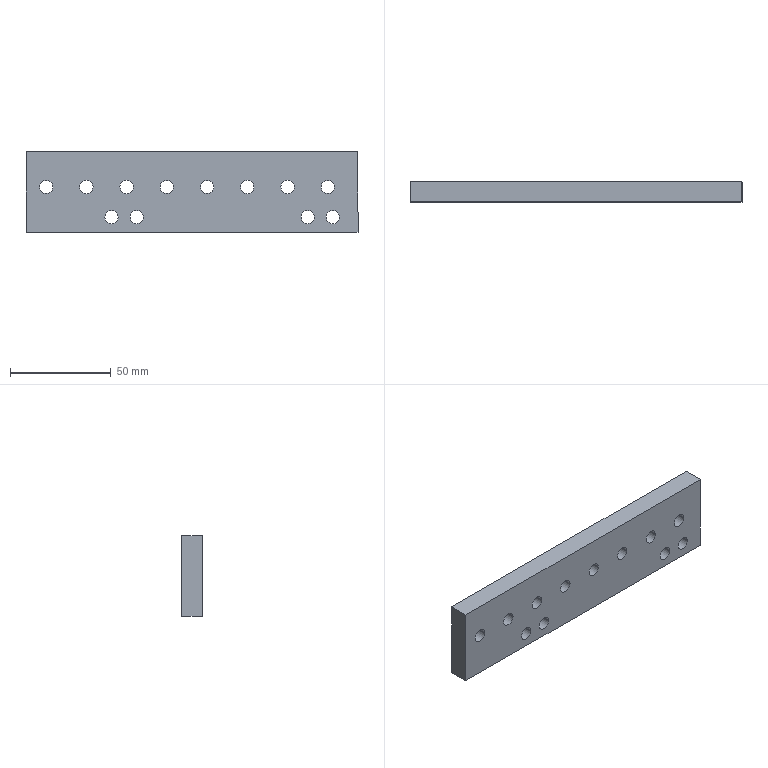Component | SolidWorks | CTM-HVS-42-02-31-4 | 1 solid | 30 faces | box 165 x 10 x 40 mm | volume 61895 mm3 | cylinder 24 | plane 6 | commonest cylinder face diameters 6.6 x24 | material Bakelite
build123d program:
from build123d import *

# Parameters (mm, degrees)
SKETCH1_W          = 185
SKETCH1_H          = 40
EXTRUDE1_DEPTH     = 10
CUT_EXTRUDE1_REACH = 152.748
SKETCH2_R          = 3.3
LPATTERN1_COUNT    = 9
LPATTERN1_PITCH    = 20
SKETCH6_W          = 20
SKETCH6_H          = 40
CUT_EXTRUDE3_DEPTH = 10


with BuildPart() as part:
    # Sketch1 → Extrude1 (new body)
    with BuildSketch(Plane.XY):
        with Locations((52.5, -20)):
            Rectangle(SKETCH1_W, SKETCH1_H)
    extrude(amount=EXTRUDE1_DEPTH)

    # Sketch2 → Cut-Extrude1 (cut, up to next)
    with BuildSketch(Plane.XY.offset(10), mode=Mode.PRIVATE) as cut_extrude1_sk1:
        with Locations((-15, -7.5)):
            Circle(SKETCH2_R)
    cut_extrude1_tool1 = extrude(cut_extrude1_sk1.sketch, amount=-CUT_EXTRUDE1_REACH, mode=Mode.PRIVATE) & part.part
    # Sketch2 → Cut-Extrude1 (cut, up to next)
    with BuildSketch(Plane.XY.offset(10), mode=Mode.PRIVATE) as cut_extrude1_sk2:
        with Locations((70, -7.5)):
            Circle(SKETCH2_R)
    cut_extrude1_tool2 = extrude(cut_extrude1_sk2.sketch, amount=-CUT_EXTRUDE1_REACH, mode=Mode.PRIVATE) & part.part
    # Sketch2 → Cut-Extrude1 (cut, up to next)
    with BuildSketch(Plane.XY.offset(10), mode=Mode.PRIVATE) as cut_extrude1_sk3:
        with Locations((-27.5, -7.5)):
            Circle(SKETCH2_R)
    cut_extrude1_tool3 = extrude(cut_extrude1_sk3.sketch, amount=-CUT_EXTRUDE1_REACH, mode=Mode.PRIVATE) & part.part
    # Sketch2 → Cut-Extrude1 (cut, up to next)
    with BuildSketch(Plane.XY.offset(10), mode=Mode.PRIVATE) as cut_extrude1_sk4:
        with Locations((82.5, -7.5)):
            Circle(SKETCH2_R)
    cut_extrude1_tool4 = extrude(cut_extrude1_sk4.sketch, amount=-CUT_EXTRUDE1_REACH, mode=Mode.PRIVATE) & part.part
    add(cut_extrude1_tool1.solids().sort_by_distance((-15, -7.5, 10))[0], mode=Mode.SUBTRACT)
    add(cut_extrude1_tool2.solids().sort_by_distance((70, -7.5, 10))[0], mode=Mode.SUBTRACT)
    add(cut_extrude1_tool3.solids().sort_by_distance((-27.5, -7.5, 10))[0], mode=Mode.SUBTRACT)
    add(cut_extrude1_tool4.solids().sort_by_distance((82.5, -7.5, 10))[0], mode=Mode.SUBTRACT)

    # Sketch4 → M6 Clearance Hole1 (revolve, cut)
    with BuildSketch(Plane(origin=(-25, -22.5, 10), x_dir=(0, -1, 0), z_dir=(1, 0, 0))):
        Polygon((0, 0), (0, 31.983), (3.3, 30), (3.3, 0), align=None)
    m6_clearance_hole1 = revolve(axis=Axis((-25, -22.5, 16.35), (0, 0, -1)), mode=Mode.SUBTRACT)

    # LPattern1: M6 Clearance Hole1 ×9
    with Locations(*[(i * LPATTERN1_PITCH, 0, 0) for i in range(1, LPATTERN1_COUNT)]):
        add(m6_clearance_hole1, mode=Mode.SUBTRACT)

    # Sketch6 → Cut-Extrude3 (cut)
    with BuildSketch(Plane.XY.offset(10)):
        with Locations((135, -20)):
            Rectangle(SKETCH6_W, SKETCH6_H)
    extrude(amount=-CUT_EXTRUDE3_DEPTH, mode=Mode.SUBTRACT)


solid = part.part

# Placed as in the assembly
solid = solid.moved(Location((275.193, -64.557, -7.5), (90, 0, -180)))
STEP:
#1=COLOUR_RGB('',0.7922,0.8196,0.9333);
#2=FILL_AREA_STYLE_COLOUR('',#1);
#3=FILL_AREA_STYLE('',(#2));
#4=SURFACE_STYLE_FILL_AREA(#3);
#5=SURFACE_SIDE_STYLE('',(#4));
#6=SURFACE_STYLE_USAGE(.BOTH.,#5);
#7=PRESENTATION_STYLE_ASSIGNMENT((#6));
#8=CARTESIAN_POINT('',(6.177,-2.542,0.5906));
#9=VERTEX_POINT('',#8);
#10=CARTESIAN_POINT('',(6.437,-2.542,0.5906));
#11=VERTEX_POINT('',#10);
#12=CARTESIAN_POINT('',(6.307,-2.542,0.5906));
#13=DIRECTION('',(-0.,1.,-0.));
#14=DIRECTION('',(1.,0.,0.));
#15=AXIS2_PLACEMENT_3D('',#12,#13,#14);
#16=CIRCLE('',#15,0.1299);
#17=EDGE_CURVE('',#9,#11,#16,.T.);
#18=ORIENTED_EDGE('',*,*,#17,.T.);
#19=CARTESIAN_POINT('',(6.437,-2.935,0.5906));
#20=VERTEX_POINT('',#19);
#21=CARTESIAN_POINT('',(6.437,-2.935,0.5906));
#22=DIRECTION('',(0.,-1.,0.));
#23=VECTOR('',#22,39.37);
#24=LINE('',#21,#23);
#25=EDGE_CURVE('',#11,#20,#24,.T.);
#26=ORIENTED_EDGE('',*,*,#25,.T.);
#27=CARTESIAN_POINT('',(6.177,-2.935,0.5906));
#28=VERTEX_POINT('',#27);
#29=CARTESIAN_POINT('',(6.307,-2.935,0.5906));
#30=DIRECTION('',(0.,-1.,0.));
#31=DIRECTION('',(-1.,0.,-0.));
#32=AXIS2_PLACEMENT_3D('',#29,#30,#31);
#33=CIRCLE('',#32,0.1299);
#34=EDGE_CURVE('',#20,#28,#33,.T.);
#35=ORIENTED_EDGE('',*,*,#34,.T.);
#36=CARTESIAN_POINT('',(6.177,-2.935,0.5906));
#37=DIRECTION('',(0.,-1.,0.));
#38=VECTOR('',#37,39.37);
#39=LINE('',#36,#38);
#40=EDGE_CURVE('',#9,#28,#39,.T.);
#41=ORIENTED_EDGE('',*,*,#40,.F.);
#42=EDGE_LOOP('',(#18,#26,#35,#41));
#43=FACE_OUTER_BOUND('',#42,.T.);
#44=CARTESIAN_POINT('',(6.307,-2.935,0.5906));
#45=DIRECTION('',(0.,-1.,0.));
#46=DIRECTION('',(-1.,0.,-0.));
#47=AXIS2_PLACEMENT_3D('',#44,#45,#46);
#48=CYLINDRICAL_SURFACE('',#47,0.1299);
#49=ADVANCED_FACE('',(#43),#48,.F.);
#50=CARTESIAN_POINT('',(6.964,-2.542,0.5906));
#51=VERTEX_POINT('',#50);
#52=CARTESIAN_POINT('',(7.224,-2.542,0.5906));
#53=VERTEX_POINT('',#52);
#54=CARTESIAN_POINT('',(7.094,-2.542,0.5906));
#55=DIRECTION('',(-0.,1.,-0.));
#56=DIRECTION('',(1.,0.,0.));
#57=AXIS2_PLACEMENT_3D('',#54,#55,#56);
#58=CIRCLE('',#57,0.1299);
#59=EDGE_CURVE('',#51,#53,#58,.T.);
#60=ORIENTED_EDGE('',*,*,#59,.T.);
#61=CARTESIAN_POINT('',(7.224,-2.935,0.5906));
#62=VERTEX_POINT('',#61);
#63=CARTESIAN_POINT('',(7.224,-2.935,0.5906));
#64=DIRECTION('',(0.,-1.,0.));
#65=VECTOR('',#64,39.37);
#66=LINE('',#63,#65);
#67=EDGE_CURVE('',#53,#62,#66,.T.);
#68=ORIENTED_EDGE('',*,*,#67,.T.);
#69=CARTESIAN_POINT('',(6.964,-2.935,0.5906));
#70=VERTEX_POINT('',#69);
#71=CARTESIAN_POINT('',(7.094,-2.935,0.5906));
#72=DIRECTION('',(0.,-1.,0.));
#73=DIRECTION('',(-1.,0.,-0.));
#74=AXIS2_PLACEMENT_3D('',#71,#72,#73);
#75=CIRCLE('',#74,0.1299);
#76=EDGE_CURVE('',#62,#70,#75,.T.);
#77=ORIENTED_EDGE('',*,*,#76,.T.);
#78=CARTESIAN_POINT('',(6.964,-2.935,0.5906));
#79=DIRECTION('',(0.,-1.,0.));
#80=VECTOR('',#79,39.37);
#81=LINE('',#78,#80);
#82=EDGE_CURVE('',#51,#70,#81,.T.);
#83=ORIENTED_EDGE('',*,*,#82,.F.);
#84=EDGE_LOOP('',(#60,#68,#77,#83));
#85=FACE_OUTER_BOUND('',#84,.T.);
#86=CARTESIAN_POINT('',(7.094,-2.935,0.5906));
#87=DIRECTION('',(0.,-1.,0.));
#88=DIRECTION('',(-1.,0.,-0.));
#89=AXIS2_PLACEMENT_3D('',#86,#87,#88);
#90=CYLINDRICAL_SURFACE('',#89,0.1299);
#91=ADVANCED_FACE('',(#85),#90,.F.);
#92=CARTESIAN_POINT('',(7.752,-2.542,0.5906));
#93=VERTEX_POINT('',#92);
#94=CARTESIAN_POINT('',(8.012,-2.542,0.5906));
#95=VERTEX_POINT('',#94);
#96=CARTESIAN_POINT('',(7.882,-2.542,0.5906));
#97=DIRECTION('',(-0.,1.,-0.));
#98=DIRECTION('',(1.,0.,0.));
#99=AXIS2_PLACEMENT_3D('',#96,#97,#98);
#100=CIRCLE('',#99,0.1299);
#101=EDGE_CURVE('',#93,#95,#100,.T.);
#102=ORIENTED_EDGE('',*,*,#101,.T.);
#103=CARTESIAN_POINT('',(8.012,-2.935,0.5906));
#104=VERTEX_POINT('',#103);
#105=CARTESIAN_POINT('',(8.012,-2.935,0.5906));
#106=DIRECTION('',(0.,-1.,0.));
#107=VECTOR('',#106,39.37);
#108=LINE('',#105,#107);
#109=EDGE_CURVE('',#95,#104,#108,.T.);
#110=ORIENTED_EDGE('',*,*,#109,.T.);
#111=CARTESIAN_POINT('',(7.752,-2.935,0.5906));
#112=VERTEX_POINT('',#111);
#113=CARTESIAN_POINT('',(7.882,-2.935,0.5906));
#114=DIRECTION('',(0.,-1.,0.));
#115=DIRECTION('',(-1.,0.,-0.));
#116=AXIS2_PLACEMENT_3D('',#113,#114,#115);
#117=CIRCLE('',#116,0.1299);
#118=EDGE_CURVE('',#104,#112,#117,.T.);
#119=ORIENTED_EDGE('',*,*,#118,.T.);
#120=CARTESIAN_POINT('',(7.752,-2.935,0.5906));
#121=DIRECTION('',(0.,-1.,0.));
#122=VECTOR('',#121,39.37);
#123=LINE('',#120,#122);
#124=EDGE_CURVE('',#93,#112,#123,.T.);
#125=ORIENTED_EDGE('',*,*,#124,.F.);
#126=EDGE_LOOP('',(#102,#110,#119,#125));
#127=FACE_OUTER_BOUND('',#126,.T.);
#128=CARTESIAN_POINT('',(7.882,-2.935,0.5906));
#129=DIRECTION('',(0.,-1.,0.));
#130=DIRECTION('',(-1.,0.,-0.));
#131=AXIS2_PLACEMENT_3D('',#128,#129,#130);
#132=CYLINDRICAL_SURFACE('',#131,0.1299);
#133=ADVANCED_FACE('',(#127),#132,.F.);
#134=CARTESIAN_POINT('',(8.539,-2.542,0.5906));
#135=VERTEX_POINT('',#134);
#136=CARTESIAN_POINT('',(8.799,-2.542,0.5906));
#137=VERTEX_POINT('',#136);
#138=CARTESIAN_POINT('',(8.669,-2.542,0.5906));
#139=DIRECTION('',(-0.,1.,-0.));
#140=DIRECTION('',(1.,0.,0.));
#141=AXIS2_PLACEMENT_3D('',#138,#139,#140);
#142=CIRCLE('',#141,0.1299);
#143=EDGE_CURVE('',#135,#137,#142,.T.);
#144=ORIENTED_EDGE('',*,*,#143,.T.);
#145=CARTESIAN_POINT('',(8.799,-2.935,0.5906));
#146=VERTEX_POINT('',#145);
#147=CARTESIAN_POINT('',(8.799,-2.935,0.5906));
#148=DIRECTION('',(0.,-1.,0.));
#149=VECTOR('',#148,39.37);
#150=LINE('',#147,#149);
#151=EDGE_CURVE('',#137,#146,#150,.T.);
#152=ORIENTED_EDGE('',*,*,#151,.T.);
#153=CARTESIAN_POINT('',(8.539,-2.935,0.5906));
#154=VERTEX_POINT('',#153);
#155=CARTESIAN_POINT('',(8.669,-2.935,0.5906));
#156=DIRECTION('',(0.,-1.,0.));
#157=DIRECTION('',(-1.,0.,-0.));
#158=AXIS2_PLACEMENT_3D('',#155,#156,#157);
#159=CIRCLE('',#158,0.1299);
#160=EDGE_CURVE('',#146,#154,#159,.T.);
#161=ORIENTED_EDGE('',*,*,#160,.T.);
#162=CARTESIAN_POINT('',(8.539,-2.935,0.5906));
#163=DIRECTION('',(0.,-1.,0.));
#164=VECTOR('',#163,39.37);
#165=LINE('',#162,#164);
#166=EDGE_CURVE('',#135,#154,#165,.T.);
#167=ORIENTED_EDGE('',*,*,#166,.F.);
#168=EDGE_LOOP('',(#144,#152,#161,#167));
#169=FACE_OUTER_BOUND('',#168,.T.);
#170=CARTESIAN_POINT('',(8.669,-2.935,0.5906));
#171=DIRECTION('',(0.,-1.,0.));
#172=DIRECTION('',(-1.,0.,-0.));
#173=AXIS2_PLACEMENT_3D('',#170,#171,#172);
#174=CYLINDRICAL_SURFACE('',#173,0.1299);
#175=ADVANCED_FACE('',(#169),#174,.F.);
#176=CARTESIAN_POINT('',(9.326,-2.542,0.5906));
#177=VERTEX_POINT('',#176);
#178=CARTESIAN_POINT('',(9.586,-2.542,0.5906));
#179=VERTEX_POINT('',#178);
#180=CARTESIAN_POINT('',(9.456,-2.542,0.5906));
#181=DIRECTION('',(-0.,1.,-0.));
#182=DIRECTION('',(1.,0.,0.));
#183=AXIS2_PLACEMENT_3D('',#180,#181,#182);
#184=CIRCLE('',#183,0.1299);
#185=EDGE_CURVE('',#177,#179,#184,.T.);
#186=ORIENTED_EDGE('',*,*,#185,.T.);
#187=CARTESIAN_POINT('',(9.586,-2.935,0.5906));
#188=VERTEX_POINT('',#187);
#189=CARTESIAN_POINT('',(9.586,-2.935,0.5906));
#190=DIRECTION('',(0.,-1.,0.));
#191=VECTOR('',#190,39.37);
#192=LINE('',#189,#191);
#193=EDGE_CURVE('',#179,#188,#192,.T.);
#194=ORIENTED_EDGE('',*,*,#193,.T.);
#195=CARTESIAN_POINT('',(9.326,-2.935,0.5906));
#196=VERTEX_POINT('',#195);
#197=CARTESIAN_POINT('',(9.456,-2.935,0.5906));
#198=DIRECTION('',(0.,-1.,0.));
#199=DIRECTION('',(-1.,0.,-0.));
#200=AXIS2_PLACEMENT_3D('',#197,#198,#199);
#201=CIRCLE('',#200,0.1299);
#202=EDGE_CURVE('',#188,#196,#201,.T.);
#203=ORIENTED_EDGE('',*,*,#202,.T.);
#204=CARTESIAN_POINT('',(9.326,-2.935,0.5906));
#205=DIRECTION('',(0.,-1.,0.));
#206=VECTOR('',#205,39.37);
#207=LINE('',#204,#206);
#208=EDGE_CURVE('',#177,#196,#207,.T.);
#209=ORIENTED_EDGE('',*,*,#208,.F.);
#210=EDGE_LOOP('',(#186,#194,#203,#209));
#211=FACE_OUTER_BOUND('',#210,.T.);
#212=CARTESIAN_POINT('',(9.456,-2.935,0.5906));
#213=DIRECTION('',(0.,-1.,0.));
#214=DIRECTION('',(-1.,0.,-0.));
#215=AXIS2_PLACEMENT_3D('',#212,#213,#214);
#216=CYLINDRICAL_SURFACE('',#215,0.1299);
#217=ADVANCED_FACE('',(#211),#216,.F.);
#218=CARTESIAN_POINT('',(10.114,-2.542,0.5906));
#219=VERTEX_POINT('',#218);
#220=CARTESIAN_POINT('',(10.374,-2.542,0.5906));
#221=VERTEX_POINT('',#220);
#222=CARTESIAN_POINT('',(10.244,-2.542,0.5906));
#223=DIRECTION('',(-0.,1.,-0.));
#224=DIRECTION('',(1.,0.,0.));
#225=AXIS2_PLACEMENT_3D('',#222,#223,#224);
#226=CIRCLE('',#225,0.1299);
#227=EDGE_CURVE('',#219,#221,#226,.T.);
#228=ORIENTED_EDGE('',*,*,#227,.T.);
#229=CARTESIAN_POINT('',(10.374,-2.935,0.5906));
#230=VERTEX_POINT('',#229);
#231=CARTESIAN_POINT('',(10.374,-2.935,0.5906));
#232=DIRECTION('',(0.,-1.,0.));
#233=VECTOR('',#232,39.37);
#234=LINE('',#231,#233);
#235=EDGE_CURVE('',#221,#230,#234,.T.);
#236=ORIENTED_EDGE('',*,*,#235,.T.);
#237=CARTESIAN_POINT('',(10.114,-2.935,0.5906));
#238=VERTEX_POINT('',#237);
#239=CARTESIAN_POINT('',(10.244,-2.935,0.5906));
#240=DIRECTION('',(0.,-1.,0.));
#241=DIRECTION('',(-1.,0.,-0.));
#242=AXIS2_PLACEMENT_3D('',#239,#240,#241);
#243=CIRCLE('',#242,0.1299);
#244=EDGE_CURVE('',#230,#238,#243,.T.);
#245=ORIENTED_EDGE('',*,*,#244,.T.);
#246=CARTESIAN_POINT('',(10.114,-2.935,0.5906));
#247=DIRECTION('',(0.,-1.,0.));
#248=VECTOR('',#247,39.37);
#249=LINE('',#246,#248);
#250=EDGE_CURVE('',#219,#238,#249,.T.);
#251=ORIENTED_EDGE('',*,*,#250,.F.);
#252=EDGE_LOOP('',(#228,#236,#245,#251));
#253=FACE_OUTER_BOUND('',#252,.T.);
#254=CARTESIAN_POINT('',(10.244,-2.935,0.5906));
#255=DIRECTION('',(0.,-1.,0.));
#256=DIRECTION('',(-1.,0.,-0.));
#257=AXIS2_PLACEMENT_3D('',#254,#255,#256);
#258=CYLINDRICAL_SURFACE('',#257,0.1299);
#259=ADVANCED_FACE('',(#253),#258,.F.);
#260=CARTESIAN_POINT('',(10.901,-2.542,0.5906));
#261=VERTEX_POINT('',#260);
#262=CARTESIAN_POINT('',(11.161,-2.542,0.5906));
#263=VERTEX_POINT('',#262);
#264=CARTESIAN_POINT('',(11.031,-2.542,0.5906));
#265=DIRECTION('',(-0.,1.,-0.));
#266=DIRECTION('',(1.,0.,0.));
#267=AXIS2_PLACEMENT_3D('',#264,#265,#266);
#268=CIRCLE('',#267,0.1299);
#269=EDGE_CURVE('',#261,#263,#268,.T.);
#270=ORIENTED_EDGE('',*,*,#269,.T.);
#271=CARTESIAN_POINT('',(11.161,-2.935,0.5906));
#272=VERTEX_POINT('',#271);
#273=CARTESIAN_POINT('',(11.161,-2.935,0.5906));
#274=DIRECTION('',(0.,-1.,0.));
#275=VECTOR('',#274,39.37);
#276=LINE('',#273,#275);
#277=EDGE_CURVE('',#263,#272,#276,.T.);
#278=ORIENTED_EDGE('',*,*,#277,.T.);
#279=CARTESIAN_POINT('',(10.901,-2.935,0.5906));
#280=VERTEX_POINT('',#279);
#281=CARTESIAN_POINT('',(11.031,-2.935,0.5906));
#282=DIRECTION('',(0.,-1.,0.));
#283=DIRECTION('',(-1.,0.,-0.));
#284=AXIS2_PLACEMENT_3D('',#281,#282,#283);
#285=CIRCLE('',#284,0.1299);
#286=EDGE_CURVE('',#272,#280,#285,.T.);
#287=ORIENTED_EDGE('',*,*,#286,.T.);
#288=CARTESIAN_POINT('',(10.901,-2.935,0.5906));
#289=DIRECTION('',(0.,-1.,0.));
#290=VECTOR('',#289,39.37);
#291=LINE('',#288,#290);
#292=EDGE_CURVE('',#261,#280,#291,.T.);
#293=ORIENTED_EDGE('',*,*,#292,.F.);
#294=EDGE_LOOP('',(#270,#278,#287,#293));
#295=FACE_OUTER_BOUND('',#294,.T.);
#296=CARTESIAN_POINT('',(11.031,-2.935,0.5906));
#297=DIRECTION('',(0.,-1.,0.));
#298=DIRECTION('',(-1.,0.,-0.));
#299=AXIS2_PLACEMENT_3D('',#296,#297,#298);
#300=CYLINDRICAL_SURFACE('',#299,0.1299);
#301=ADVANCED_FACE('',(#295),#300,.F.);
#302=CARTESIAN_POINT('',(11.689,-2.542,0.5906));
#303=VERTEX_POINT('',#302);
#304=CARTESIAN_POINT('',(11.949,-2.542,0.5906));
#305=VERTEX_POINT('',#304);
#306=CARTESIAN_POINT('',(11.819,-2.542,0.5906));
#307=DIRECTION('',(-0.,1.,-0.));
#308=DIRECTION('',(1.,0.,0.));
#309=AXIS2_PLACEMENT_3D('',#306,#307,#308);
#310=CIRCLE('',#309,0.1299);
#311=EDGE_CURVE('',#303,#305,#310,.T.);
#312=ORIENTED_EDGE('',*,*,#311,.T.);
#313=CARTESIAN_POINT('',(11.949,-2.935,0.5906));
#314=VERTEX_POINT('',#313);
#315=CARTESIAN_POINT('',(11.949,-2.935,0.5906));
#316=DIRECTION('',(0.,-1.,0.));
#317=VECTOR('',#316,39.37);
#318=LINE('',#315,#317);
#319=EDGE_CURVE('',#305,#314,#318,.T.);
#320=ORIENTED_EDGE('',*,*,#319,.T.);
#321=CARTESIAN_POINT('',(11.689,-2.935,0.5906));
#322=VERTEX_POINT('',#321);
#323=CARTESIAN_POINT('',(11.819,-2.935,0.5906));
#324=DIRECTION('',(0.,-1.,0.));
#325=DIRECTION('',(-1.,0.,-0.));
#326=AXIS2_PLACEMENT_3D('',#323,#324,#325);
#327=CIRCLE('',#326,0.1299);
#328=EDGE_CURVE('',#314,#322,#327,.T.);
#329=ORIENTED_EDGE('',*,*,#328,.T.);
#330=CARTESIAN_POINT('',(11.689,-2.935,0.5906));
#331=DIRECTION('',(0.,-1.,0.));
#332=VECTOR('',#331,39.37);
#333=LINE('',#330,#332);
#334=EDGE_CURVE('',#303,#322,#333,.T.);
#335=ORIENTED_EDGE('',*,*,#334,.F.);
#336=EDGE_LOOP('',(#312,#320,#329,#335));
#337=FACE_OUTER_BOUND('',#336,.T.);
#338=CARTESIAN_POINT('',(11.819,-2.935,0.5906));
#339=DIRECTION('',(0.,-1.,0.));
#340=DIRECTION('',(-1.,0.,-0.));
#341=AXIS2_PLACEMENT_3D('',#338,#339,#340);
#342=CYLINDRICAL_SURFACE('',#341,0.1299);
#343=ADVANCED_FACE('',(#337),#342,.F.);
#344=CARTESIAN_POINT('',(7.716,-2.542,0.));
#345=VERTEX_POINT('',#344);
#346=CARTESIAN_POINT('',(7.456,-2.542,0.));
#347=VERTEX_POINT('',#346);
#348=CARTESIAN_POINT('',(7.586,-2.542,0.));
#349=DIRECTION('',(0.,-1.,0.));
#350=DIRECTION('',(1.,0.,0.));
#351=AXIS2_PLACEMENT_3D('',#348,#349,#350);
#352=CIRCLE('',#351,0.1299);
#353=EDGE_CURVE('',#345,#347,#352,.T.);
#354=ORIENTED_EDGE('',*,*,#353,.F.);
#355=CARTESIAN_POINT('',(7.716,-2.935,0.));
#356=VERTEX_POINT('',#355);
#357=CARTESIAN_POINT('',(7.716,-2.542,0.));
#358=DIRECTION('',(0.,-1.,0.));
#359=VECTOR('',#358,39.37);
#360=LINE('',#357,#359);
#361=EDGE_CURVE('',#345,#356,#360,.T.);
#362=ORIENTED_EDGE('',*,*,#361,.T.);
#363=CARTESIAN_POINT('',(7.456,-2.935,0.));
#364=VERTEX_POINT('',#363);
#365=CARTESIAN_POINT('',(7.586,-2.935,0.));
#366=DIRECTION('',(0.,-1.,0.));
#367=DIRECTION('',(-1.,0.,-0.));
#368=AXIS2_PLACEMENT_3D('',#365,#366,#367);
#369=CIRCLE('',#368,0.1299);
#370=EDGE_CURVE('',#356,#364,#369,.T.);
#371=ORIENTED_EDGE('',*,*,#370,.T.);
#372=CARTESIAN_POINT('',(7.456,-2.542,0.));
#373=DIRECTION('',(0.,-1.,0.));
#374=VECTOR('',#373,39.37);
#375=LINE('',#372,#374);
#376=EDGE_CURVE('',#347,#364,#375,.T.);
#377=ORIENTED_EDGE('',*,*,#376,.F.);
#378=EDGE_LOOP('',(#354,#362,#371,#377));
#379=FACE_OUTER_BOUND('',#378,.T.);
#380=CARTESIAN_POINT('',(7.586,-2.542,0.));
#381=DIRECTION('',(0.,-1.,0.));
#382=DIRECTION('',(-1.,0.,-0.));
#383=AXIS2_PLACEMENT_3D('',#380,#381,#382);
#384=CYLINDRICAL_SURFACE('',#383,0.1299);
#385=ADVANCED_FACE('',(#379),#384,.F.);
#386=CARTESIAN_POINT('',(12.047,-2.542,0.));
#387=VERTEX_POINT('',#386);
#388=CARTESIAN_POINT('',(11.787,-2.542,0.));
#389=VERTEX_POINT('',#388);
#390=CARTESIAN_POINT('',(11.917,-2.542,0.));
#391=DIRECTION('',(0.,-1.,0.));
#392=DIRECTION('',(1.,0.,0.));
#393=AXIS2_PLACEMENT_3D('',#390,#391,#392);
#394=CIRCLE('',#393,0.1299);
#395=EDGE_CURVE('',#387,#389,#394,.T.);
#396=ORIENTED_EDGE('',*,*,#395,.F.);
#397=CARTESIAN_POINT('',(12.047,-2.935,0.));
#398=VERTEX_POINT('',#397);
#399=CARTESIAN_POINT('',(12.047,-2.542,0.));
#400=DIRECTION('',(0.,-1.,0.));
#401=VECTOR('',#400,39.37);
#402=LINE('',#399,#401);
#403=EDGE_CURVE('',#387,#398,#402,.T.);
#404=ORIENTED_EDGE('',*,*,#403,.T.);
#405=CARTESIAN_POINT('',(11.787,-2.935,0.));
#406=VERTEX_POINT('',#405);
#407=CARTESIAN_POINT('',(11.917,-2.935,0.));
#408=DIRECTION('',(0.,-1.,0.));
#409=DIRECTION('',(-1.,0.,-0.));
#410=AXIS2_PLACEMENT_3D('',#407,#408,#409);
#411=CIRCLE('',#410,0.1299);
#412=EDGE_CURVE('',#398,#406,#411,.T.);
#413=ORIENTED_EDGE('',*,*,#412,.T.);
#414=CARTESIAN_POINT('',(11.787,-2.542,0.));
#415=DIRECTION('',(0.,-1.,0.));
#416=VECTOR('',#415,39.37);
#417=LINE('',#414,#416);
#418=EDGE_CURVE('',#389,#406,#417,.T.);
#419=ORIENTED_EDGE('',*,*,#418,.F.);
#420=EDGE_LOOP('',(#396,#404,#413,#419));
#421=FACE_OUTER_BOUND('',#420,.T.);
#422=CARTESIAN_POINT('',(11.917,-2.542,0.));
#423=DIRECTION('',(0.,-1.,0.));
#424=DIRECTION('',(-1.,0.,-0.));
#425=AXIS2_PLACEMENT_3D('',#422,#423,#424);
#426=CYLINDRICAL_SURFACE('',#425,0.1299);
#427=ADVANCED_FACE('',(#421),#426,.F.);
#428=CARTESIAN_POINT('',(8.208,-2.542,0.));
#429=VERTEX_POINT('',#428);
#430=CARTESIAN_POINT('',(7.949,-2.542,0.));
#431=VERTEX_POINT('',#430);
#432=CARTESIAN_POINT('',(8.078,-2.542,0.));
#433=DIRECTION('',(0.,-1.,0.));
#434=DIRECTION('',(1.,0.,0.));
#435=AXIS2_PLACEMENT_3D('',#432,#433,#434);
#436=CIRCLE('',#435,0.1299);
#437=EDGE_CURVE('',#429,#431,#436,.T.);
#438=ORIENTED_EDGE('',*,*,#437,.F.);
#439=CARTESIAN_POINT('',(8.208,-2.935,0.));
#440=VERTEX_POINT('',#439);
#441=CARTESIAN_POINT('',(8.208,-2.542,0.));
#442=DIRECTION('',(0.,-1.,0.));
#443=VECTOR('',#442,39.37);
#444=LINE('',#441,#443);
#445=EDGE_CURVE('',#429,#440,#444,.T.);
#446=ORIENTED_EDGE('',*,*,#445,.T.);
#447=CARTESIAN_POINT('',(7.949,-2.935,0.));
#448=VERTEX_POINT('',#447);
#449=CARTESIAN_POINT('',(8.078,-2.935,0.));
#450=DIRECTION('',(0.,-1.,0.));
#451=DIRECTION('',(-1.,0.,-0.));
#452=AXIS2_PLACEMENT_3D('',#449,#450,#451);
#453=CIRCLE('',#452,0.1299);
#454=EDGE_CURVE('',#440,#448,#453,.T.);
#455=ORIENTED_EDGE('',*,*,#454,.T.);
#456=CARTESIAN_POINT('',(7.949,-2.542,0.));
#457=DIRECTION('',(0.,-1.,0.));
#458=VECTOR('',#457,39.37);
#459=LINE('',#456,#458);
#460=EDGE_CURVE('',#431,#448,#459,.T.);
#461=ORIENTED_EDGE('',*,*,#460,.F.);
#462=EDGE_LOOP('',(#438,#446,#455,#461));
#463=FACE_OUTER_BOUND('',#462,.T.);
#464=CARTESIAN_POINT('',(8.078,-2.542,0.));
#465=DIRECTION('',(0.,-1.,0.));
#466=DIRECTION('',(-1.,0.,-0.));
#467=AXIS2_PLACEMENT_3D('',#464,#465,#466);
#468=CYLINDRICAL_SURFACE('',#467,0.1299);
#469=ADVANCED_FACE('',(#463),#468,.F.);
#470=CARTESIAN_POINT('',(11.555,-2.542,0.));
#471=VERTEX_POINT('',#470);
#472=CARTESIAN_POINT('',(11.295,-2.542,0.));
#473=VERTEX_POINT('',#472);
#474=CARTESIAN_POINT('',(11.425,-2.542,0.));
#475=DIRECTION('',(0.,-1.,0.));
#476=DIRECTION('',(1.,0.,0.));
#477=AXIS2_PLACEMENT_3D('',#474,#475,#476);
#478=CIRCLE('',#477,0.1299);
#479=EDGE_CURVE('',#471,#473,#478,.T.);
#480=ORIENTED_EDGE('',*,*,#479,.F.);
#481=CARTESIAN_POINT('',(11.555,-2.935,0.));
#482=VERTEX_POINT('',#481);
#483=CARTESIAN_POINT('',(11.555,-2.542,0.));
#484=DIRECTION('',(0.,-1.,0.));
#485=VECTOR('',#484,39.37);
#486=LINE('',#483,#485);
#487=EDGE_CURVE('',#471,#482,#486,.T.);
#488=ORIENTED_EDGE('',*,*,#487,.T.);
#489=CARTESIAN_POINT('',(11.295,-2.935,0.));
#490=VERTEX_POINT('',#489);
#491=CARTESIAN_POINT('',(11.425,-2.935,0.));
#492=DIRECTION('',(0.,-1.,0.));
#493=DIRECTION('',(-1.,0.,-0.));
#494=AXIS2_PLACEMENT_3D('',#491,#492,#493);
#495=CIRCLE('',#494,0.1299);
#496=EDGE_CURVE('',#482,#490,#495,.T.);
#497=ORIENTED_EDGE('',*,*,#496,.T.);
#498=CARTESIAN_POINT('',(11.295,-2.542,0.));
#499=DIRECTION('',(0.,-1.,0.));
#500=VECTOR('',#499,39.37);
#501=LINE('',#498,#500);
#502=EDGE_CURVE('',#473,#490,#501,.T.);
#503=ORIENTED_EDGE('',*,*,#502,.F.);
#504=EDGE_LOOP('',(#480,#488,#497,#503));
#505=FACE_OUTER_BOUND('',#504,.T.);
#506=CARTESIAN_POINT('',(11.425,-2.542,0.));
#507=DIRECTION('',(0.,-1.,0.));
#508=DIRECTION('',(-1.,0.,-0.));
#509=AXIS2_PLACEMENT_3D('',#506,#507,#508);
#510=CYLINDRICAL_SURFACE('',#509,0.1299);
#511=ADVANCED_FACE('',(#505),#510,.F.);
#512=CARTESIAN_POINT('',(12.409,-2.542,1.28));
#513=VERTEX_POINT('',#512);
#514=CARTESIAN_POINT('',(5.913,-2.542,1.28));
#515=VERTEX_POINT('',#514);
#516=CARTESIAN_POINT('',(12.409,-2.542,1.28));
#517=DIRECTION('',(-1.,-0.,-0.));
#518=VECTOR('',#517,39.37);
#519=LINE('',#516,#518);
#520=EDGE_CURVE('',#513,#515,#519,.T.);
#521=ORIENTED_EDGE('',*,*,#520,.T.);
#522=CARTESIAN_POINT('',(5.913,-2.935,1.28));
#523=VERTEX_POINT('',#522);
#524=CARTESIAN_POINT('',(5.913,-2.542,1.28));
#525=DIRECTION('',(0.,-1.,0.));
#526=VECTOR('',#525,39.37);
#527=LINE('',#524,#526);
#528=EDGE_CURVE('',#515,#523,#527,.T.);
#529=ORIENTED_EDGE('',*,*,#528,.T.);
#530=CARTESIAN_POINT('',(12.409,-2.935,1.28));
#531=VERTEX_POINT('',#530);
#532=CARTESIAN_POINT('',(12.409,-2.935,1.28));
#533=DIRECTION('',(-1.,-0.,-0.));
#534=VECTOR('',#533,39.37);
#535=LINE('',#532,#534);
#536=EDGE_CURVE('',#531,#523,#535,.T.);
#537=ORIENTED_EDGE('',*,*,#536,.F.);
#538=CARTESIAN_POINT('',(12.409,-2.935,1.28));
#539=DIRECTION('',(-0.,1.,-0.));
#540=VECTOR('',#539,39.37);
#541=LINE('',#538,#540);
#542=EDGE_CURVE('',#531,#513,#541,.T.);
#543=ORIENTED_EDGE('',*,*,#542,.T.);
#544=EDGE_LOOP('',(#521,#529,#537,#543));
#545=FACE_OUTER_BOUND('',#544,.T.);
#546=CARTESIAN_POINT('',(12.409,-2.935,1.28));
#547=DIRECTION('',(0.,-0.,-1.));
#548=DIRECTION('',(0.,-1.,0.));
#549=AXIS2_PLACEMENT_3D('',#546,#547,#548);
#550=PLANE('',#549);
#551=ADVANCED_FACE('',(#545),#550,.F.);
#552=CARTESIAN_POINT('',(5.913,-2.935,-0.2953));
#553=VERTEX_POINT('',#552);
#554=CARTESIAN_POINT('',(12.409,-2.935,-0.2953));
#555=VERTEX_POINT('',#554);
#556=CARTESIAN_POINT('',(12.409,-2.935,-0.2953));
#557=DIRECTION('',(1.,0.,0.));
#558=VECTOR('',#557,39.37);
#559=LINE('',#556,#558);
#560=EDGE_CURVE('',#553,#555,#559,.T.);
#561=ORIENTED_EDGE('',*,*,#560,.F.);
#562=CARTESIAN_POINT('',(5.913,-2.542,-0.2953));
#563=VERTEX_POINT('',#562);
#564=CARTESIAN_POINT('',(5.913,-2.542,-0.2953));
#565=DIRECTION('',(0.,-1.,0.));
#566=VECTOR('',#565,39.37);
#567=LINE('',#564,#566);
#568=EDGE_CURVE('',#563,#553,#567,.T.);
#569=ORIENTED_EDGE('',*,*,#568,.F.);
#570=CARTESIAN_POINT('',(12.409,-2.542,-0.2953));
#571=VERTEX_POINT('',#570);
#572=CARTESIAN_POINT('',(12.409,-2.542,-0.2953));
#573=DIRECTION('',(1.,0.,0.));
#574=VECTOR('',#573,39.37);
#575=LINE('',#572,#574);
#576=EDGE_CURVE('',#563,#571,#575,.T.);
#577=ORIENTED_EDGE('',*,*,#576,.T.);
#578=CARTESIAN_POINT('',(12.409,-2.935,-0.2953));
#579=DIRECTION('',(-0.,1.,-0.));
#580=VECTOR('',#579,39.37);
#581=LINE('',#578,#580);
#582=EDGE_CURVE('',#555,#571,#581,.T.);
#583=ORIENTED_EDGE('',*,*,#582,.F.);
#584=EDGE_LOOP('',(#561,#569,#577,#583));
#585=FACE_OUTER_BOUND('',#584,.T.);
#586=CARTESIAN_POINT('',(12.409,-2.935,-0.2953));
#587=DIRECTION('',(-0.,0.,1.));
#588=DIRECTION('',(-0.,1.,-0.));
#589=AXIS2_PLACEMENT_3D('',#586,#587,#588);
#590=PLANE('',#589);
#591=ADVANCED_FACE('',(#585),#590,.F.);
#592=CARTESIAN_POINT('',(12.409,-2.542,-0.2953));
#593=DIRECTION('',(-0.,0.,1.));
#594=VECTOR('',#593,39.37);
#595=LINE('',#592,#594);
#596=EDGE_CURVE('',#571,#513,#595,.T.);
#597=ORIENTED_EDGE('',*,*,#596,.T.);
#598=ORIENTED_EDGE('',*,*,#542,.F.);
#599=CARTESIAN_POINT('',(12.409,-2.935,-0.2953));
#600=DIRECTION('',(-0.,0.,1.));
#601=VECTOR('',#600,39.37);
#602=LINE('',#599,#601);
#603=EDGE_CURVE('',#555,#531,#602,.T.);
#604=ORIENTED_EDGE('',*,*,#603,.F.);
#605=ORIENTED_EDGE('',*,*,#582,.T.);
#606=EDGE_LOOP('',(#597,#598,#604,#605));
#607=FACE_OUTER_BOUND('',#606,.T.);
#608=CARTESIAN_POINT('',(12.409,-2.935,-0.2953));
#609=DIRECTION('',(-1.,-0.,-0.));
#610=DIRECTION('',(-0.,1.,-0.));
#611=AXIS2_PLACEMENT_3D('',#608,#609,#610);
#612=PLANE('',#611);
#613=ADVANCED_FACE('',(#607),#612,.F.);
#614=CARTESIAN_POINT('',(11.031,-2.935,0.5906));
#615=DIRECTION('',(0.,-1.,0.));
#616=DIRECTION('',(-1.,0.,-0.));
#617=AXIS2_PLACEMENT_3D('',#614,#615,#616);
#618=CIRCLE('',#617,0.1299);
#619=EDGE_CURVE('',#280,#272,#618,.T.);
#620=ORIENTED_EDGE('',*,*,#619,.F.);
#621=ORIENTED_EDGE('',*,*,#286,.F.);
#622=EDGE_LOOP('',(#620,#621));
#623=FACE_BOUND('',#622,.T.);
#624=CARTESIAN_POINT('',(11.819,-2.935,0.5906));
#625=DIRECTION('',(0.,-1.,0.));
#626=DIRECTION('',(-1.,0.,-0.));
#627=AXIS2_PLACEMENT_3D('',#624,#625,#626);
#628=CIRCLE('',#627,0.1299);
#629=EDGE_CURVE('',#322,#314,#628,.T.);
#630=ORIENTED_EDGE('',*,*,#629,.F.);
#631=ORIENTED_EDGE('',*,*,#328,.F.);
#632=EDGE_LOOP('',(#630,#631));
#633=FACE_BOUND('',#632,.T.);
#634=CARTESIAN_POINT('',(7.586,-2.935,0.));
#635=DIRECTION('',(0.,-1.,0.));
#636=DIRECTION('',(-1.,0.,-0.));
#637=AXIS2_PLACEMENT_3D('',#634,#635,#636);
#638=CIRCLE('',#637,0.1299);
#639=EDGE_CURVE('',#364,#356,#638,.T.);
#640=ORIENTED_EDGE('',*,*,#639,.F.);
#641=ORIENTED_EDGE('',*,*,#370,.F.);
#642=EDGE_LOOP('',(#640,#641));
#643=FACE_BOUND('',#642,.T.);
#644=CARTESIAN_POINT('',(11.917,-2.935,0.));
#645=DIRECTION('',(0.,-1.,0.));
#646=DIRECTION('',(-1.,0.,-0.));
#647=AXIS2_PLACEMENT_3D('',#644,#645,#646);
#648=CIRCLE('',#647,0.1299);
#649=EDGE_CURVE('',#406,#398,#648,.T.);
#650=ORIENTED_EDGE('',*,*,#649,.F.);
#651=ORIENTED_EDGE('',*,*,#412,.F.);
#652=EDGE_LOOP('',(#650,#651));
#653=FACE_BOUND('',#652,.T.);
#654=CARTESIAN_POINT('',(8.078,-2.935,0.));
#655=DIRECTION('',(0.,-1.,0.));
#656=DIRECTION('',(-1.,0.,-0.));
#657=AXIS2_PLACEMENT_3D('',#654,#655,#656);
#658=CIRCLE('',#657,0.1299);
#659=EDGE_CURVE('',#448,#440,#658,.T.);
#660=ORIENTED_EDGE('',*,*,#659,.F.);
#661=ORIENTED_EDGE('',*,*,#454,.F.);
#662=EDGE_LOOP('',(#660,#661));
#663=FACE_BOUND('',#662,.T.);
#664=CARTESIAN_POINT('',(11.425,-2.935,0.));
#665=DIRECTION('',(0.,-1.,0.));
#666=DIRECTION('',(-1.,0.,-0.));
#667=AXIS2_PLACEMENT_3D('',#664,#665,#666);
#668=CIRCLE('',#667,0.1299);
#669=EDGE_CURVE('',#490,#482,#668,.T.);
#670=ORIENTED_EDGE('',*,*,#669,.F.);
#671=ORIENTED_EDGE('',*,*,#496,.F.);
#672=EDGE_LOOP('',(#670,#671));
#673=FACE_BOUND('',#672,.T.);
#674=ORIENTED_EDGE('',*,*,#536,.T.);
#675=CARTESIAN_POINT('',(5.913,-2.935,-0.2953));
#676=DIRECTION('',(-0.,0.,1.));
#677=VECTOR('',#676,39.37);
#678=LINE('',#675,#677);
#679=EDGE_CURVE('',#553,#523,#678,.T.);
#680=ORIENTED_EDGE('',*,*,#679,.F.);
#681=ORIENTED_EDGE('',*,*,#560,.T.);
#682=ORIENTED_EDGE('',*,*,#603,.T.);
#683=EDGE_LOOP('',(#674,#680,#681,#682));
#684=FACE_OUTER_BOUND('',#683,.T.);
#685=CARTESIAN_POINT('',(10.244,-2.935,0.5906));
#686=DIRECTION('',(0.,-1.,0.));
#687=DIRECTION('',(-1.,0.,-0.));
#688=AXIS2_PLACEMENT_3D('',#685,#686,#687);
#689=CIRCLE('',#688,0.1299);
#690=EDGE_CURVE('',#238,#230,#689,.T.);
#691=ORIENTED_EDGE('',*,*,#690,.F.);
#692=ORIENTED_EDGE('',*,*,#244,.F.);
#693=EDGE_LOOP('',(#691,#692));
#694=FACE_BOUND('',#693,.T.);
#695=CARTESIAN_POINT('',(9.456,-2.935,0.5906));
#696=DIRECTION('',(0.,-1.,0.));
#697=DIRECTION('',(-1.,0.,-0.));
#698=AXIS2_PLACEMENT_3D('',#695,#696,#697);
#699=CIRCLE('',#698,0.1299);
#700=EDGE_CURVE('',#196,#188,#699,.T.);
#701=ORIENTED_EDGE('',*,*,#700,.F.);
#702=ORIENTED_EDGE('',*,*,#202,.F.);
#703=EDGE_LOOP('',(#701,#702));
#704=FACE_BOUND('',#703,.T.);
#705=CARTESIAN_POINT('',(8.669,-2.935,0.5906));
#706=DIRECTION('',(0.,-1.,0.));
#707=DIRECTION('',(-1.,0.,-0.));
#708=AXIS2_PLACEMENT_3D('',#705,#706,#707);
#709=CIRCLE('',#708,0.1299);
#710=EDGE_CURVE('',#154,#146,#709,.T.);
#711=ORIENTED_EDGE('',*,*,#710,.F.);
#712=ORIENTED_EDGE('',*,*,#160,.F.);
#713=EDGE_LOOP('',(#711,#712));
#714=FACE_BOUND('',#713,.T.);
#715=CARTESIAN_POINT('',(7.882,-2.935,0.5906));
#716=DIRECTION('',(0.,-1.,0.));
#717=DIRECTION('',(-1.,0.,-0.));
#718=AXIS2_PLACEMENT_3D('',#715,#716,#717);
#719=CIRCLE('',#718,0.1299);
#720=EDGE_CURVE('',#112,#104,#719,.T.);
#721=ORIENTED_EDGE('',*,*,#720,.F.);
#722=ORIENTED_EDGE('',*,*,#118,.F.);
#723=EDGE_LOOP('',(#721,#722));
#724=FACE_BOUND('',#723,.T.);
#725=CARTESIAN_POINT('',(7.094,-2.935,0.5906));
#726=DIRECTION('',(0.,-1.,0.));
#727=DIRECTION('',(-1.,0.,-0.));
#728=AXIS2_PLACEMENT_3D('',#725,#726,#727);
#729=CIRCLE('',#728,0.1299);
#730=EDGE_CURVE('',#70,#62,#729,.T.);
#731=ORIENTED_EDGE('',*,*,#730,.F.);
#732=ORIENTED_EDGE('',*,*,#76,.F.);
#733=EDGE_LOOP('',(#731,#732));
#734=FACE_BOUND('',#733,.T.);
#735=CARTESIAN_POINT('',(6.307,-2.935,0.5906));
#736=DIRECTION('',(0.,-1.,0.));
#737=DIRECTION('',(-1.,0.,-0.));
#738=AXIS2_PLACEMENT_3D('',#735,#736,#737);
#739=CIRCLE('',#738,0.1299);
#740=EDGE_CURVE('',#28,#20,#739,.T.);
#741=ORIENTED_EDGE('',*,*,#740,.F.);
#742=ORIENTED_EDGE('',*,*,#34,.F.);
#743=EDGE_LOOP('',(#741,#742));
#744=FACE_BOUND('',#743,.T.);
#745=CARTESIAN_POINT('',(5.126,-2.935,1.28));
#746=DIRECTION('',(-0.,1.,-0.));
#747=DIRECTION('',(1.,0.,0.));
#748=AXIS2_PLACEMENT_3D('',#745,#746,#747);
#749=PLANE('',#748);
#750=ADVANCED_FACE('',(#623,#633,#643,#653,#663,#673,#684,#694,#704,#714,#724,#734,#744),#749,.F.);
#751=CARTESIAN_POINT('',(5.913,-2.542,-0.2953));
#752=DIRECTION('',(-0.,0.,1.));
#753=VECTOR('',#752,39.37);
#754=LINE('',#751,#753);
#755=EDGE_CURVE('',#563,#515,#754,.T.);
#756=ORIENTED_EDGE('',*,*,#755,.T.);
#757=ORIENTED_EDGE('',*,*,#520,.F.);
#758=ORIENTED_EDGE('',*,*,#596,.F.);
#759=ORIENTED_EDGE('',*,*,#576,.F.);
#760=EDGE_LOOP('',(#756,#757,#758,#759));
#761=FACE_OUTER_BOUND('',#760,.T.);
#762=ORIENTED_EDGE('',*,*,#269,.F.);
#763=CARTESIAN_POINT('',(11.031,-2.542,0.5906));
#764=DIRECTION('',(-0.,1.,-0.));
#765=DIRECTION('',(1.,0.,0.));
#766=AXIS2_PLACEMENT_3D('',#763,#764,#765);
#767=CIRCLE('',#766,0.1299);
#768=EDGE_CURVE('',#263,#261,#767,.T.);
#769=ORIENTED_EDGE('',*,*,#768,.F.);
#770=EDGE_LOOP('',(#762,#769));
#771=FACE_BOUND('',#770,.T.);
#772=ORIENTED_EDGE('',*,*,#311,.F.);
#773=CARTESIAN_POINT('',(11.819,-2.542,0.5906));
#774=DIRECTION('',(-0.,1.,-0.));
#775=DIRECTION('',(1.,0.,0.));
#776=AXIS2_PLACEMENT_3D('',#773,#774,#775);
#777=CIRCLE('',#776,0.1299);
#778=EDGE_CURVE('',#305,#303,#777,.T.);
#779=ORIENTED_EDGE('',*,*,#778,.F.);
#780=EDGE_LOOP('',(#772,#779));
#781=FACE_BOUND('',#780,.T.);
#782=CARTESIAN_POINT('',(7.586,-2.542,0.));
#783=DIRECTION('',(0.,-1.,0.));
#784=DIRECTION('',(1.,0.,0.));
#785=AXIS2_PLACEMENT_3D('',#782,#783,#784);
#786=CIRCLE('',#785,0.1299);
#787=EDGE_CURVE('',#347,#345,#786,.T.);
#788=ORIENTED_EDGE('',*,*,#787,.T.);
#789=ORIENTED_EDGE('',*,*,#353,.T.);
#790=EDGE_LOOP('',(#788,#789));
#791=FACE_BOUND('',#790,.T.);
#792=CARTESIAN_POINT('',(11.917,-2.542,0.));
#793=DIRECTION('',(0.,-1.,0.));
#794=DIRECTION('',(1.,0.,0.));
#795=AXIS2_PLACEMENT_3D('',#792,#793,#794);
#796=CIRCLE('',#795,0.1299);
#797=EDGE_CURVE('',#389,#387,#796,.T.);
#798=ORIENTED_EDGE('',*,*,#797,.T.);
#799=ORIENTED_EDGE('',*,*,#395,.T.);
#800=EDGE_LOOP('',(#798,#799));
#801=FACE_BOUND('',#800,.T.);
#802=CARTESIAN_POINT('',(8.078,-2.542,0.));
#803=DIRECTION('',(0.,-1.,0.));
#804=DIRECTION('',(1.,0.,0.));
#805=AXIS2_PLACEMENT_3D('',#802,#803,#804);
#806=CIRCLE('',#805,0.1299);
#807=EDGE_CURVE('',#431,#429,#806,.T.);
#808=ORIENTED_EDGE('',*,*,#807,.T.);
#809=ORIENTED_EDGE('',*,*,#437,.T.);
#810=EDGE_LOOP('',(#808,#809));
#811=FACE_BOUND('',#810,.T.);
#812=CARTESIAN_POINT('',(11.425,-2.542,0.));
#813=DIRECTION('',(0.,-1.,0.));
#814=DIRECTION('',(1.,0.,0.));
#815=AXIS2_PLACEMENT_3D('',#812,#813,#814);
#816=CIRCLE('',#815,0.1299);
#817=EDGE_CURVE('',#473,#471,#816,.T.);
#818=ORIENTED_EDGE('',*,*,#817,.T.);
#819=ORIENTED_EDGE('',*,*,#479,.T.);
#820=EDGE_LOOP('',(#818,#819));
#821=FACE_BOUND('',#820,.T.);
#822=ORIENTED_EDGE('',*,*,#227,.F.);
#823=CARTESIAN_POINT('',(10.244,-2.542,0.5906));
#824=DIRECTION('',(-0.,1.,-0.));
#825=DIRECTION('',(1.,0.,0.));
#826=AXIS2_PLACEMENT_3D('',#823,#824,#825);
#827=CIRCLE('',#826,0.1299);
#828=EDGE_CURVE('',#221,#219,#827,.T.);
#829=ORIENTED_EDGE('',*,*,#828,.F.);
#830=EDGE_LOOP('',(#822,#829));
#831=FACE_BOUND('',#830,.T.);
#832=ORIENTED_EDGE('',*,*,#185,.F.);
#833=CARTESIAN_POINT('',(9.456,-2.542,0.5906));
#834=DIRECTION('',(-0.,1.,-0.));
#835=DIRECTION('',(1.,0.,0.));
#836=AXIS2_PLACEMENT_3D('',#833,#834,#835);
#837=CIRCLE('',#836,0.1299);
#838=EDGE_CURVE('',#179,#177,#837,.T.);
#839=ORIENTED_EDGE('',*,*,#838,.F.);
#840=EDGE_LOOP('',(#832,#839));
#841=FACE_BOUND('',#840,.T.);
#842=ORIENTED_EDGE('',*,*,#143,.F.);
#843=CARTESIAN_POINT('',(8.669,-2.542,0.5906));
#844=DIRECTION('',(-0.,1.,-0.));
#845=DIRECTION('',(1.,0.,0.));
#846=AXIS2_PLACEMENT_3D('',#843,#844,#845);
#847=CIRCLE('',#846,0.1299);
#848=EDGE_CURVE('',#137,#135,#847,.T.);
#849=ORIENTED_EDGE('',*,*,#848,.F.);
#850=EDGE_LOOP('',(#842,#849));
#851=FACE_BOUND('',#850,.T.);
#852=ORIENTED_EDGE('',*,*,#101,.F.);
#853=CARTESIAN_POINT('',(7.882,-2.542,0.5906));
#854=DIRECTION('',(-0.,1.,-0.));
#855=DIRECTION('',(1.,0.,0.));
#856=AXIS2_PLACEMENT_3D('',#853,#854,#855);
#857=CIRCLE('',#856,0.1299);
#858=EDGE_CURVE('',#95,#93,#857,.T.);
#859=ORIENTED_EDGE('',*,*,#858,.F.);
#860=EDGE_LOOP('',(#852,#859));
#861=FACE_BOUND('',#860,.T.);
#862=ORIENTED_EDGE('',*,*,#59,.F.);
#863=CARTESIAN_POINT('',(7.094,-2.542,0.5906));
#864=DIRECTION('',(-0.,1.,-0.));
#865=DIRECTION('',(1.,0.,0.));
#866=AXIS2_PLACEMENT_3D('',#863,#864,#865);
#867=CIRCLE('',#866,0.1299);
#868=EDGE_CURVE('',#53,#51,#867,.T.);
#869=ORIENTED_EDGE('',*,*,#868,.F.);
#870=EDGE_LOOP('',(#862,#869));
#871=FACE_BOUND('',#870,.T.);
#872=ORIENTED_EDGE('',*,*,#17,.F.);
#873=CARTESIAN_POINT('',(6.307,-2.542,0.5906));
#874=DIRECTION('',(-0.,1.,-0.));
#875=DIRECTION('',(1.,0.,0.));
#876=AXIS2_PLACEMENT_3D('',#873,#874,#875);
#877=CIRCLE('',#876,0.1299);
#878=EDGE_CURVE('',#11,#9,#877,.T.);
#879=ORIENTED_EDGE('',*,*,#878,.F.);
#880=EDGE_LOOP('',(#872,#879));
#881=FACE_BOUND('',#880,.T.);
#882=CARTESIAN_POINT('',(5.126,-2.542,1.28));
#883=DIRECTION('',(-0.,1.,-0.));
#884=DIRECTION('',(1.,0.,0.));
#885=AXIS2_PLACEMENT_3D('',#882,#883,#884);
#886=PLANE('',#885);
#887=ADVANCED_FACE('',(#761,#771,#781,#791,#801,#811,#821,#831,#841,#851,#861,#871,#881),#886,.T.);
#888=ORIENTED_EDGE('',*,*,#487,.F.);
#889=ORIENTED_EDGE('',*,*,#817,.F.);
#890=ORIENTED_EDGE('',*,*,#502,.T.);
#891=ORIENTED_EDGE('',*,*,#669,.T.);
#892=EDGE_LOOP('',(#888,#889,#890,#891));
#893=FACE_OUTER_BOUND('',#892,.T.);
#894=CARTESIAN_POINT('',(11.425,-2.542,0.));
#895=DIRECTION('',(0.,-1.,0.));
#896=DIRECTION('',(-1.,0.,-0.));
#897=AXIS2_PLACEMENT_3D('',#894,#895,#896);
#898=CYLINDRICAL_SURFACE('',#897,0.1299);
#899=ADVANCED_FACE('',(#893),#898,.F.);
#900=ORIENTED_EDGE('',*,*,#445,.F.);
#901=ORIENTED_EDGE('',*,*,#807,.F.);
#902=ORIENTED_EDGE('',*,*,#460,.T.);
#903=ORIENTED_EDGE('',*,*,#659,.T.);
#904=EDGE_LOOP('',(#900,#901,#902,#903));
#905=FACE_OUTER_BOUND('',#904,.T.);
#906=CARTESIAN_POINT('',(8.078,-2.542,0.));
#907=DIRECTION('',(0.,-1.,0.));
#908=DIRECTION('',(-1.,0.,-0.));
#909=AXIS2_PLACEMENT_3D('',#906,#907,#908);
#910=CYLINDRICAL_SURFACE('',#909,0.1299);
#911=ADVANCED_FACE('',(#905),#910,.F.);
#912=ORIENTED_EDGE('',*,*,#403,.F.);
#913=ORIENTED_EDGE('',*,*,#797,.F.);
#914=ORIENTED_EDGE('',*,*,#418,.T.);
#915=ORIENTED_EDGE('',*,*,#649,.T.);
#916=EDGE_LOOP('',(#912,#913,#914,#915));
#917=FACE_OUTER_BOUND('',#916,.T.);
#918=CARTESIAN_POINT('',(11.917,-2.542,0.));
#919=DIRECTION('',(0.,-1.,0.));
#920=DIRECTION('',(-1.,0.,-0.));
#921=AXIS2_PLACEMENT_3D('',#918,#919,#920);
#922=CYLINDRICAL_SURFACE('',#921,0.1299);
#923=ADVANCED_FACE('',(#917),#922,.F.);
#924=ORIENTED_EDGE('',*,*,#361,.F.);
#925=ORIENTED_EDGE('',*,*,#787,.F.);
#926=ORIENTED_EDGE('',*,*,#376,.T.);
#927=ORIENTED_EDGE('',*,*,#639,.T.);
#928=EDGE_LOOP('',(#924,#925,#926,#927));
#929=FACE_OUTER_BOUND('',#928,.T.);
#930=CARTESIAN_POINT('',(7.586,-2.542,0.));
#931=DIRECTION('',(0.,-1.,0.));
#932=DIRECTION('',(-1.,0.,-0.));
#933=AXIS2_PLACEMENT_3D('',#930,#931,#932);
#934=CYLINDRICAL_SURFACE('',#933,0.1299);
#935=ADVANCED_FACE('',(#929),#934,.F.);
#936=ORIENTED_EDGE('',*,*,#319,.F.);
#937=ORIENTED_EDGE('',*,*,#778,.T.);
#938=ORIENTED_EDGE('',*,*,#334,.T.);
#939=ORIENTED_EDGE('',*,*,#629,.T.);
#940=EDGE_LOOP('',(#936,#937,#938,#939));
#941=FACE_OUTER_BOUND('',#940,.T.);
#942=CARTESIAN_POINT('',(11.819,-2.935,0.5906));
#943=DIRECTION('',(0.,-1.,0.));
#944=DIRECTION('',(-1.,0.,-0.));
#945=AXIS2_PLACEMENT_3D('',#942,#943,#944);
#946=CYLINDRICAL_SURFACE('',#945,0.1299);
#947=ADVANCED_FACE('',(#941),#946,.F.);
#948=ORIENTED_EDGE('',*,*,#277,.F.);
#949=ORIENTED_EDGE('',*,*,#768,.T.);
#950=ORIENTED_EDGE('',*,*,#292,.T.);
#951=ORIENTED_EDGE('',*,*,#619,.T.);
#952=EDGE_LOOP('',(#948,#949,#950,#951));
#953=FACE_OUTER_BOUND('',#952,.T.);
#954=CARTESIAN_POINT('',(11.031,-2.935,0.5906));
#955=DIRECTION('',(0.,-1.,0.));
#956=DIRECTION('',(-1.,0.,-0.));
#957=AXIS2_PLACEMENT_3D('',#954,#955,#956);
#958=CYLINDRICAL_SURFACE('',#957,0.1299);
#959=ADVANCED_FACE('',(#953),#958,.F.);
#960=ORIENTED_EDGE('',*,*,#235,.F.);
#961=ORIENTED_EDGE('',*,*,#828,.T.);
#962=ORIENTED_EDGE('',*,*,#250,.T.);
#963=ORIENTED_EDGE('',*,*,#690,.T.);
#964=EDGE_LOOP('',(#960,#961,#962,#963));
#965=FACE_OUTER_BOUND('',#964,.T.);
#966=CARTESIAN_POINT('',(10.244,-2.935,0.5906));
#967=DIRECTION('',(0.,-1.,0.));
#968=DIRECTION('',(-1.,0.,-0.));
#969=AXIS2_PLACEMENT_3D('',#966,#967,#968);
#970=CYLINDRICAL_SURFACE('',#969,0.1299);
#971=ADVANCED_FACE('',(#965),#970,.F.);
#972=ORIENTED_EDGE('',*,*,#193,.F.);
#973=ORIENTED_EDGE('',*,*,#838,.T.);
#974=ORIENTED_EDGE('',*,*,#208,.T.);
#975=ORIENTED_EDGE('',*,*,#700,.T.);
#976=EDGE_LOOP('',(#972,#973,#974,#975));
#977=FACE_OUTER_BOUND('',#976,.T.);
#978=CARTESIAN_POINT('',(9.456,-2.935,0.5906));
#979=DIRECTION('',(0.,-1.,0.));
#980=DIRECTION('',(-1.,0.,-0.));
#981=AXIS2_PLACEMENT_3D('',#978,#979,#980);
#982=CYLINDRICAL_SURFACE('',#981,0.1299);
#983=ADVANCED_FACE('',(#977),#982,.F.);
#984=ORIENTED_EDGE('',*,*,#151,.F.);
#985=ORIENTED_EDGE('',*,*,#848,.T.);
#986=ORIENTED_EDGE('',*,*,#166,.T.);
#987=ORIENTED_EDGE('',*,*,#710,.T.);
#988=EDGE_LOOP('',(#984,#985,#986,#987));
#989=FACE_OUTER_BOUND('',#988,.T.);
#990=CARTESIAN_POINT('',(8.669,-2.935,0.5906));
#991=DIRECTION('',(0.,-1.,0.));
#992=DIRECTION('',(-1.,0.,-0.));
#993=AXIS2_PLACEMENT_3D('',#990,#991,#992);
#994=CYLINDRICAL_SURFACE('',#993,0.1299);
#995=ADVANCED_FACE('',(#989),#994,.F.);
#996=ORIENTED_EDGE('',*,*,#109,.F.);
#997=ORIENTED_EDGE('',*,*,#858,.T.);
#998=ORIENTED_EDGE('',*,*,#124,.T.);
#999=ORIENTED_EDGE('',*,*,#720,.T.);
#1000=EDGE_LOOP('',(#996,#997,#998,#999));
#1001=FACE_OUTER_BOUND('',#1000,.T.);
#1002=CARTESIAN_POINT('',(7.882,-2.935,0.5906));
#1003=DIRECTION('',(0.,-1.,0.));
#1004=DIRECTION('',(-1.,0.,-0.));
#1005=AXIS2_PLACEMENT_3D('',#1002,#1003,#1004);
#1006=CYLINDRICAL_SURFACE('',#1005,0.1299);
#1007=ADVANCED_FACE('',(#1001),#1006,.F.);
#1008=ORIENTED_EDGE('',*,*,#67,.F.);
#1009=ORIENTED_EDGE('',*,*,#868,.T.);
#1010=ORIENTED_EDGE('',*,*,#82,.T.);
#1011=ORIENTED_EDGE('',*,*,#730,.T.);
#1012=EDGE_LOOP('',(#1008,#1009,#1010,#1011));
#1013=FACE_OUTER_BOUND('',#1012,.T.);
#1014=CARTESIAN_POINT('',(7.094,-2.935,0.5906));
#1015=DIRECTION('',(0.,-1.,0.));
#1016=DIRECTION('',(-1.,0.,-0.));
#1017=AXIS2_PLACEMENT_3D('',#1014,#1015,#1016);
#1018=CYLINDRICAL_SURFACE('',#1017,0.1299);
#1019=ADVANCED_FACE('',(#1013),#1018,.F.);
#1020=ORIENTED_EDGE('',*,*,#25,.F.);
#1021=ORIENTED_EDGE('',*,*,#878,.T.);
#1022=ORIENTED_EDGE('',*,*,#40,.T.);
#1023=ORIENTED_EDGE('',*,*,#740,.T.);
#1024=EDGE_LOOP('',(#1020,#1021,#1022,#1023));
#1025=FACE_OUTER_BOUND('',#1024,.T.);
#1026=CARTESIAN_POINT('',(6.307,-2.935,0.5906));
#1027=DIRECTION('',(0.,-1.,0.));
#1028=DIRECTION('',(-1.,0.,-0.));
#1029=AXIS2_PLACEMENT_3D('',#1026,#1027,#1028);
#1030=CYLINDRICAL_SURFACE('',#1029,0.1299);
#1031=ADVANCED_FACE('',(#1025),#1030,.F.);
#1032=ORIENTED_EDGE('',*,*,#679,.T.);
#1033=ORIENTED_EDGE('',*,*,#528,.F.);
#1034=ORIENTED_EDGE('',*,*,#755,.F.);
#1035=ORIENTED_EDGE('',*,*,#568,.T.);
#1036=EDGE_LOOP('',(#1032,#1033,#1034,#1035));
#1037=FACE_OUTER_BOUND('',#1036,.T.);
#1038=CARTESIAN_POINT('',(5.913,-2.542,-0.2953));
#1039=DIRECTION('',(1.,0.,0.));
#1040=DIRECTION('',(-0.,0.,1.));
#1041=AXIS2_PLACEMENT_3D('',#1038,#1039,#1040);
#1042=PLANE('',#1041);
#1043=ADVANCED_FACE('',(#1037),#1042,.F.);
#1044=CLOSED_SHELL('',(#49,#91,#133,#175,#217,#259,#301,#343,#385,#427,#469,#511,#551,#591,#613,#750,#887,#899,#911,#923,#935,#947,#959,#971,#983,#995,#1007,#1019,#1031,#1043));
#1045=MANIFOLD_SOLID_BREP('',#1044);
#1046=STYLED_ITEM('',(#7),#1045);
#1047=PRESENTATION_LAYER_ASSIGNMENT('','',(#1046));
#1048=CARTESIAN_POINT('',(0.,0.,0.));
#1049=DIRECTION('',(0.,0.,1.));
#1050=DIRECTION('',(1.,0.,0.));
#1051=AXIS2_PLACEMENT_3D('',#1048,#1049,#1050);
#1052=(LENGTH_UNIT()NAMED_UNIT(*)SI_UNIT($,.METRE.));
#1053=LENGTH_MEASURE_WITH_UNIT(LENGTH_MEASURE(0.0254),#1052);
#1054=DIMENSIONAL_EXPONENTS(1.,0.,0.,0.,0.,0.,0.);
#1055=(CONVERSION_BASED_UNIT('',#1053)LENGTH_UNIT()NAMED_UNIT(#1054));
#1056=UNCERTAINTY_MEASURE_WITH_UNIT(LENGTH_MEASURE(0.00001),#1055,'','');
#1057=(NAMED_UNIT(*)PLANE_ANGLE_UNIT()SI_UNIT($,.RADIAN.));
#1058=(NAMED_UNIT(*)SI_UNIT($,.STERADIAN.)SOLID_ANGLE_UNIT());
#1059=(GEOMETRIC_REPRESENTATION_CONTEXT(3)GLOBAL_UNCERTAINTY_ASSIGNED_CONTEXT((#1056))GLOBAL_UNIT_ASSIGNED_CONTEXT((#1055,#1057,#1058))REPRESENTATION_CONTEXT('',''));
#1060=ADVANCED_BREP_SHAPE_REPRESENTATION('',(#1045,#1051),#1059);
#1061=(LENGTH_UNIT()NAMED_UNIT(*)SI_UNIT($,.METRE.));
#1062=LENGTH_MEASURE_WITH_UNIT(LENGTH_MEASURE(0.0254),#1061);
#1063=DIMENSIONAL_EXPONENTS(1.,0.,0.,0.,0.,0.,0.);
#1064=(CONVERSION_BASED_UNIT('',#1062)LENGTH_UNIT()NAMED_UNIT(#1063));
#1065=UNCERTAINTY_MEASURE_WITH_UNIT(LENGTH_MEASURE(0.00001),#1064,'','');
#1066=(NAMED_UNIT(*)PLANE_ANGLE_UNIT()SI_UNIT($,.RADIAN.));
#1067=(NAMED_UNIT(*)SI_UNIT($,.STERADIAN.)SOLID_ANGLE_UNIT());
#1068=(GEOMETRIC_REPRESENTATION_CONTEXT(3)GLOBAL_UNCERTAINTY_ASSIGNED_CONTEXT((#1065))GLOBAL_UNIT_ASSIGNED_CONTEXT((#1064,#1066,#1067))REPRESENTATION_CONTEXT('',''));
#1069=MECHANICAL_DESIGN_GEOMETRIC_PRESENTATION_REPRESENTATION('',(#1046),#1068);